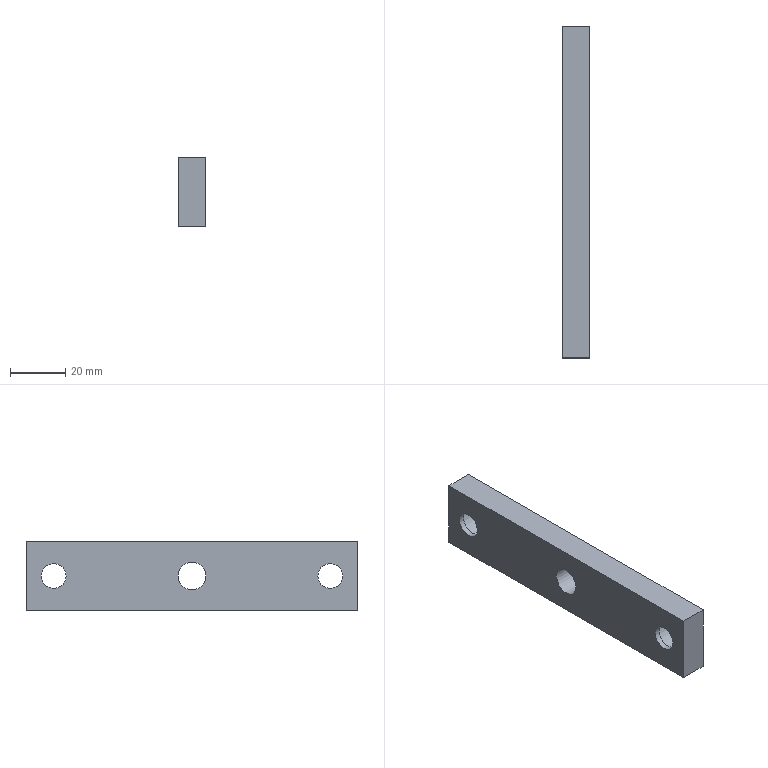Component | NX | FIXTURE_MOUNT_2 | 1 solid | 13 faces | box 10 x 120 x 25 mm | volume 26497 mm3 | plane 8 | cylinder 5 | commonest cylinder face diameters 9 x2 14 x2 10 x1
STEP:
#1=CARTESIAN_POINT('',(0.,0.,0.));
#2=DIRECTION('',(0.,0.,1.));
#3=DIRECTION('',(1.,0.,0.));
#4=AXIS2_PLACEMENT_3D('',#1,#2,#3);
#5=CARTESIAN_POINT('',(746.689,-204.802,-1307.5));
#6=VERTEX_POINT('',#5);
#7=CARTESIAN_POINT('',(746.689,-200.302,-1307.5));
#8=DIRECTION('',(-1.,0.,0.));
#9=DIRECTION('',(0.,-1.,0.));
#10=AXIS2_PLACEMENT_3D('',#7,#8,#9);
#11=CIRCLE('',#10,4.5);
#12=CARTESIAN_POINT('',(756.689,-200.302,-1307.5));
#13=DIRECTION('',(-1.,0.,0.));
#14=DIRECTION('',(0.,-1.,0.));
#15=AXIS2_PLACEMENT_3D('',#12,#13,#14);
#16=CYLINDRICAL_SURFACE('',#15,4.5);
#17=CARTESIAN_POINT('',(0.,10.));
#18=DIRECTION('',(1.,0.));
#19=VECTOR('',#18,1.);
#20=LINE('',#17,#19);
#21=(GEOMETRIC_REPRESENTATION_CONTEXT(2)PARAMETRIC_REPRESENTATION_CONTEXT()REPRESENTATION_CONTEXT('',''));
#22=DEFINITIONAL_REPRESENTATION('',(#20),#21);
#23=PCURVE('',#16,#22);
#24=CARTESIAN_POINT('',(746.689,-150.302,-1307.5));
#25=DIRECTION('',(-1.,0.,0.));
#26=DIRECTION('',(0.,-1.,0.));
#27=AXIS2_PLACEMENT_3D('',#24,#25,#26);
#28=PLANE('',#27);
#29=CARTESIAN_POINT('',(50.,0.));
#30=DIRECTION('',(1.,0.));
#31=AXIS2_PLACEMENT_2D('',#29,#30);
#32=CIRCLE('',#31,4.5);
#33=(GEOMETRIC_REPRESENTATION_CONTEXT(2)PARAMETRIC_REPRESENTATION_CONTEXT()REPRESENTATION_CONTEXT('',''));
#34=DEFINITIONAL_REPRESENTATION('',(#32),#33);
#35=PCURVE('',#28,#34);
#36=SURFACE_CURVE('',#11,(#23,#35),.PCURVE_S1.);
#37=EDGE_CURVE('',#6,#6,#36,.T.);
#38=ORIENTED_EDGE('',*,*,#37,.F.);
#39=CARTESIAN_POINT('',(748.689,-204.802,-1307.5));
#40=VERTEX_POINT('',#39);
#41=CARTESIAN_POINT('',(748.689,-204.802,-1307.5));
#42=CARTESIAN_POINT('',(746.689,-204.802,-1307.5));
#43=B_SPLINE_CURVE_WITH_KNOTS('',1,(#41,#42),.UNSPECIFIED.,.F.,.F.,(2,2),(8.,10.),.PIECEWISE_BEZIER_KNOTS.);
#44=CARTESIAN_POINT('',(0.,0.));
#45=DIRECTION('',(0.,1.));
#46=VECTOR('',#45,1.);
#47=LINE('',#44,#46);
#48=(GEOMETRIC_REPRESENTATION_CONTEXT(2)PARAMETRIC_REPRESENTATION_CONTEXT()REPRESENTATION_CONTEXT('',''));
#49=DEFINITIONAL_REPRESENTATION('',(#47),#48);
#50=PCURVE('',#16,#49);
#51=CARTESIAN_POINT('',(6.283,0.));
#52=DIRECTION('',(0.,1.));
#53=VECTOR('',#52,1.);
#54=LINE('',#51,#53);
#55=(GEOMETRIC_REPRESENTATION_CONTEXT(2)PARAMETRIC_REPRESENTATION_CONTEXT()REPRESENTATION_CONTEXT('',''));
#56=DEFINITIONAL_REPRESENTATION('',(#54),#55);
#57=PCURVE('',#16,#56);
#58=SEAM_CURVE('',#43,(#50,#57),.PCURVE_S1.);
#59=EDGE_CURVE('',#40,#6,#58,.T.);
#60=ORIENTED_EDGE('',*,*,#59,.F.);
#61=CARTESIAN_POINT('',(748.689,-195.802,-1307.5));
#62=VERTEX_POINT('',#61);
#63=CARTESIAN_POINT('',(748.689,-200.302,-1307.5));
#64=DIRECTION('',(-1.,0.,0.));
#65=DIRECTION('',(0.,1.,0.));
#66=AXIS2_PLACEMENT_3D('',#63,#64,#65);
#67=CIRCLE('',#66,4.5);
#68=CARTESIAN_POINT('',(-3.142,8.));
#69=DIRECTION('',(1.,0.));
#70=VECTOR('',#69,1.);
#71=LINE('',#68,#70);
#72=(GEOMETRIC_REPRESENTATION_CONTEXT(2)PARAMETRIC_REPRESENTATION_CONTEXT()REPRESENTATION_CONTEXT('',''));
#73=DEFINITIONAL_REPRESENTATION('',(#71),#72);
#74=PCURVE('',#16,#73);
#75=CARTESIAN_POINT('',(748.689,-200.302,-1307.5));
#76=DIRECTION('',(1.,0.,0.));
#77=DIRECTION('',(0.,1.,0.));
#78=AXIS2_PLACEMENT_3D('',#75,#76,#77);
#79=PLANE('',#78);
#80=CARTESIAN_POINT('',(4.5,0.));
#81=CARTESIAN_POINT('',(4.5,-7.794));
#82=CARTESIAN_POINT('',(-2.25,-3.897));
#83=CARTESIAN_POINT('',(-9.,-0.));
#84=CARTESIAN_POINT('',(-2.25,3.897));
#85=CARTESIAN_POINT('',(4.5,7.794));
#86=CARTESIAN_POINT('',(4.5,0.));
#87=(BOUNDED_CURVE()B_SPLINE_CURVE(2,(#80,#81,#82,#83,#84,#85,#86),.UNSPECIFIED.,.T.,.F.)B_SPLINE_CURVE_WITH_KNOTS((1,2,2,2,2,1),(-2.094,0.,2.094,4.189,6.283,8.378),.UNSPECIFIED.)CURVE()GEOMETRIC_REPRESENTATION_ITEM()RATIONAL_B_SPLINE_CURVE((1.,0.5,1.,0.5,1.,0.5,1.))REPRESENTATION_ITEM(''));
#88=(GEOMETRIC_REPRESENTATION_CONTEXT(2)PARAMETRIC_REPRESENTATION_CONTEXT()REPRESENTATION_CONTEXT('',''));
#89=DEFINITIONAL_REPRESENTATION('',(#87),#88);
#90=PCURVE('',#79,#89);
#91=SURFACE_CURVE('',#67,(#74,#90),.PCURVE_S1.);
#92=EDGE_CURVE('',#40,#62,#91,.T.);
#93=ORIENTED_EDGE('',*,*,#92,.T.);
#94=CARTESIAN_POINT('',(748.689,-200.302,-1307.5));
#95=DIRECTION('',(-1.,0.,0.));
#96=DIRECTION('',(0.,1.,0.));
#97=AXIS2_PLACEMENT_3D('',#94,#95,#96);
#98=CIRCLE('',#97,4.5);
#99=CARTESIAN_POINT('',(3.142,8.));
#100=DIRECTION('',(1.,0.));
#101=VECTOR('',#100,1.);
#102=LINE('',#99,#101);
#103=(GEOMETRIC_REPRESENTATION_CONTEXT(2)PARAMETRIC_REPRESENTATION_CONTEXT()REPRESENTATION_CONTEXT('',''));
#104=DEFINITIONAL_REPRESENTATION('',(#102),#103);
#105=PCURVE('',#16,#104);
#106=CARTESIAN_POINT('',(4.5,0.));
#107=CARTESIAN_POINT('',(4.5,-7.794));
#108=CARTESIAN_POINT('',(-2.25,-3.897));
#109=CARTESIAN_POINT('',(-9.,-0.));
#110=CARTESIAN_POINT('',(-2.25,3.897));
#111=CARTESIAN_POINT('',(4.5,7.794));
#112=CARTESIAN_POINT('',(4.5,0.));
#113=(BOUNDED_CURVE()B_SPLINE_CURVE(2,(#106,#107,#108,#109,#110,#111,#112),.UNSPECIFIED.,.T.,.F.)B_SPLINE_CURVE_WITH_KNOTS((1,2,2,2,2,1),(-2.094,0.,2.094,4.189,6.283,8.378),.UNSPECIFIED.)CURVE()GEOMETRIC_REPRESENTATION_ITEM()RATIONAL_B_SPLINE_CURVE((1.,0.5,1.,0.5,1.,0.5,1.))REPRESENTATION_ITEM(''));
#114=(GEOMETRIC_REPRESENTATION_CONTEXT(2)PARAMETRIC_REPRESENTATION_CONTEXT()REPRESENTATION_CONTEXT('',''));
#115=DEFINITIONAL_REPRESENTATION('',(#113),#114);
#116=PCURVE('',#79,#115);
#117=SURFACE_CURVE('',#98,(#105,#116),.PCURVE_S1.);
#118=EDGE_CURVE('',#62,#40,#117,.T.);
#119=ORIENTED_EDGE('',*,*,#118,.T.);
#120=ORIENTED_EDGE('',*,*,#59,.T.);
#121=EDGE_LOOP('',(#38,#60,#93,#119,#120));
#122=FACE_BOUND('',#121,.F.);
#123=ADVANCED_FACE('',(#122),#16,.F.);
#124=CARTESIAN_POINT('',(746.689,-95.802,-1307.5));
#125=VERTEX_POINT('',#124);
#126=CARTESIAN_POINT('',(746.689,-100.302,-1307.5));
#127=DIRECTION('',(1.,0.,0.));
#128=DIRECTION('',(0.,1.,0.));
#129=AXIS2_PLACEMENT_3D('',#126,#127,#128);
#130=CIRCLE('',#129,4.5);
#131=CARTESIAN_POINT('',(756.689,-100.302,-1307.5));
#132=DIRECTION('',(-1.,0.,0.));
#133=DIRECTION('',(0.,-1.,0.));
#134=AXIS2_PLACEMENT_3D('',#131,#132,#133);
#135=CYLINDRICAL_SURFACE('',#134,4.5);
#136=CARTESIAN_POINT('',(9.425,10.));
#137=DIRECTION('',(-1.,0.));
#138=VECTOR('',#137,1.);
#139=LINE('',#136,#138);
#140=(GEOMETRIC_REPRESENTATION_CONTEXT(2)PARAMETRIC_REPRESENTATION_CONTEXT()REPRESENTATION_CONTEXT('',''));
#141=DEFINITIONAL_REPRESENTATION('',(#139),#140);
#142=PCURVE('',#135,#141);
#143=CARTESIAN_POINT('',(-54.5,0.));
#144=CARTESIAN_POINT('',(-54.5,7.794));
#145=CARTESIAN_POINT('',(-47.75,3.897));
#146=CARTESIAN_POINT('',(-41.,0.));
#147=CARTESIAN_POINT('',(-47.75,-3.897));
#148=CARTESIAN_POINT('',(-54.5,-7.794));
#149=CARTESIAN_POINT('',(-54.5,0.));
#150=(BOUNDED_CURVE()B_SPLINE_CURVE(2,(#143,#144,#145,#146,#147,#148,#149),.UNSPECIFIED.,.T.,.F.)B_SPLINE_CURVE_WITH_KNOTS((1,2,2,2,2,1),(-2.094,0.,2.094,4.189,6.283,8.378),.UNSPECIFIED.)CURVE()GEOMETRIC_REPRESENTATION_ITEM()RATIONAL_B_SPLINE_CURVE((1.,0.5,1.,0.5,1.,0.5,1.))REPRESENTATION_ITEM(''));
#151=(GEOMETRIC_REPRESENTATION_CONTEXT(2)PARAMETRIC_REPRESENTATION_CONTEXT()REPRESENTATION_CONTEXT('',''));
#152=DEFINITIONAL_REPRESENTATION('',(#150),#151);
#153=PCURVE('',#28,#152);
#154=SURFACE_CURVE('',#130,(#142,#153),.PCURVE_S1.);
#155=EDGE_CURVE('',#125,#125,#154,.T.);
#156=ORIENTED_EDGE('',*,*,#155,.T.);
#157=CARTESIAN_POINT('',(748.689,-95.802,-1307.5));
#158=VERTEX_POINT('',#157);
#159=CARTESIAN_POINT('',(748.689,-95.802,-1307.5));
#160=CARTESIAN_POINT('',(746.689,-95.802,-1307.5));
#161=B_SPLINE_CURVE_WITH_KNOTS('',1,(#159,#160),.UNSPECIFIED.,.F.,.F.,(2,2),(8.,10.),.PIECEWISE_BEZIER_KNOTS.);
#162=CARTESIAN_POINT('',(3.142,0.));
#163=DIRECTION('',(0.,1.));
#164=VECTOR('',#163,1.);
#165=LINE('',#162,#164);
#166=(GEOMETRIC_REPRESENTATION_CONTEXT(2)PARAMETRIC_REPRESENTATION_CONTEXT()REPRESENTATION_CONTEXT('',''));
#167=DEFINITIONAL_REPRESENTATION('',(#165),#166);
#168=PCURVE('',#135,#167);
#169=CARTESIAN_POINT('',(9.425,0.));
#170=DIRECTION('',(0.,1.));
#171=VECTOR('',#170,1.);
#172=LINE('',#169,#171);
#173=(GEOMETRIC_REPRESENTATION_CONTEXT(2)PARAMETRIC_REPRESENTATION_CONTEXT()REPRESENTATION_CONTEXT('',''));
#174=DEFINITIONAL_REPRESENTATION('',(#172),#173);
#175=PCURVE('',#135,#174);
#176=SEAM_CURVE('',#161,(#168,#175),.PCURVE_S1.);
#177=EDGE_CURVE('',#158,#125,#176,.T.);
#178=ORIENTED_EDGE('',*,*,#177,.F.);
#179=CARTESIAN_POINT('',(748.689,-100.302,-1307.5));
#180=DIRECTION('',(1.,0.,0.));
#181=DIRECTION('',(0.,1.,0.));
#182=AXIS2_PLACEMENT_3D('',#179,#180,#181);
#183=CIRCLE('',#182,4.5);
#184=CARTESIAN_POINT('',(9.425,8.));
#185=DIRECTION('',(-1.,0.));
#186=VECTOR('',#185,1.);
#187=LINE('',#184,#186);
#188=(GEOMETRIC_REPRESENTATION_CONTEXT(2)PARAMETRIC_REPRESENTATION_CONTEXT()REPRESENTATION_CONTEXT('',''));
#189=DEFINITIONAL_REPRESENTATION('',(#187),#188);
#190=PCURVE('',#135,#189);
#191=CARTESIAN_POINT('',(748.689,-100.302,-1307.5));
#192=DIRECTION('',(1.,0.,0.));
#193=DIRECTION('',(0.,1.,0.));
#194=AXIS2_PLACEMENT_3D('',#191,#192,#193);
#195=PLANE('',#194);
#196=CARTESIAN_POINT('',(0.,0.));
#197=DIRECTION('',(1.,0.));
#198=AXIS2_PLACEMENT_2D('',#196,#197);
#199=CIRCLE('',#198,4.5);
#200=(GEOMETRIC_REPRESENTATION_CONTEXT(2)PARAMETRIC_REPRESENTATION_CONTEXT()REPRESENTATION_CONTEXT('',''));
#201=DEFINITIONAL_REPRESENTATION('',(#199),#200);
#202=PCURVE('',#195,#201);
#203=SURFACE_CURVE('',#183,(#190,#202),.PCURVE_S1.);
#204=EDGE_CURVE('',#158,#158,#203,.T.);
#205=ORIENTED_EDGE('',*,*,#204,.F.);
#206=ORIENTED_EDGE('',*,*,#177,.T.);
#207=EDGE_LOOP('',(#156,#178,#205,#206));
#208=FACE_BOUND('',#207,.F.);
#209=ADVANCED_FACE('',(#208),#135,.F.);
#210=CARTESIAN_POINT('',(746.689,-210.302,-1295.));
#211=VERTEX_POINT('',#210);
#212=CARTESIAN_POINT('',(746.689,-210.302,-1320.));
#213=VERTEX_POINT('',#212);
#214=CARTESIAN_POINT('',(746.689,-210.302,-1295.));
#215=DIRECTION('',(0.,0.,-1.));
#216=VECTOR('',#215,1.);
#217=LINE('',#214,#216);
#218=CARTESIAN_POINT('',(756.689,-210.302,-1295.));
#219=DIRECTION('',(0.,1.,0.));
#220=DIRECTION('',(-1.,0.,0.));
#221=AXIS2_PLACEMENT_3D('',#218,#219,#220);
#222=PLANE('',#221);
#223=CARTESIAN_POINT('',(10.,0.));
#224=DIRECTION('',(0.,-1.));
#225=VECTOR('',#224,1.);
#226=LINE('',#223,#225);
#227=(GEOMETRIC_REPRESENTATION_CONTEXT(2)PARAMETRIC_REPRESENTATION_CONTEXT()REPRESENTATION_CONTEXT('',''));
#228=DEFINITIONAL_REPRESENTATION('',(#226),#227);
#229=PCURVE('',#222,#228);
#230=CARTESIAN_POINT('',(60.,12.5));
#231=DIRECTION('',(0.,-1.));
#232=VECTOR('',#231,1.);
#233=LINE('',#230,#232);
#234=(GEOMETRIC_REPRESENTATION_CONTEXT(2)PARAMETRIC_REPRESENTATION_CONTEXT()REPRESENTATION_CONTEXT('',''));
#235=DEFINITIONAL_REPRESENTATION('',(#233),#234);
#236=PCURVE('',#28,#235);
#237=SURFACE_CURVE('',#217,(#229,#236),.PCURVE_S1.);
#238=EDGE_CURVE('',#211,#213,#237,.T.);
#239=ORIENTED_EDGE('',*,*,#238,.T.);
#240=CARTESIAN_POINT('',(756.689,-210.302,-1320.));
#241=VERTEX_POINT('',#240);
#242=CARTESIAN_POINT('',(756.689,-210.302,-1320.));
#243=DIRECTION('',(-1.,0.,0.));
#244=VECTOR('',#243,1.);
#245=LINE('',#242,#244);
#246=CARTESIAN_POINT('',(0.,-25.));
#247=DIRECTION('',(1.,0.));
#248=VECTOR('',#247,1.);
#249=LINE('',#246,#248);
#250=(GEOMETRIC_REPRESENTATION_CONTEXT(2)PARAMETRIC_REPRESENTATION_CONTEXT()REPRESENTATION_CONTEXT('',''));
#251=DEFINITIONAL_REPRESENTATION('',(#249),#250);
#252=PCURVE('',#222,#251);
#253=CARTESIAN_POINT('',(756.689,-210.302,-1320.));
#254=DIRECTION('',(0.,0.,1.));
#255=DIRECTION('',(1.,0.,0.));
#256=AXIS2_PLACEMENT_3D('',#253,#254,#255);
#257=PLANE('',#256);
#258=CARTESIAN_POINT('',(0.,0.));
#259=DIRECTION('',(-1.,0.));
#260=VECTOR('',#259,1.);
#261=LINE('',#258,#260);
#262=(GEOMETRIC_REPRESENTATION_CONTEXT(2)PARAMETRIC_REPRESENTATION_CONTEXT()REPRESENTATION_CONTEXT('',''));
#263=DEFINITIONAL_REPRESENTATION('',(#261),#262);
#264=PCURVE('',#257,#263);
#265=SURFACE_CURVE('',#245,(#252,#264),.PCURVE_S1.);
#266=EDGE_CURVE('',#241,#213,#265,.T.);
#267=ORIENTED_EDGE('',*,*,#266,.F.);
#268=CARTESIAN_POINT('',(756.689,-210.302,-1295.));
#269=VERTEX_POINT('',#268);
#270=CARTESIAN_POINT('',(756.689,-210.302,-1295.));
#271=DIRECTION('',(0.,0.,-1.));
#272=VECTOR('',#271,1.);
#273=LINE('',#270,#272);
#274=CARTESIAN_POINT('',(0.,0.));
#275=DIRECTION('',(0.,-1.));
#276=VECTOR('',#275,1.);
#277=LINE('',#274,#276);
#278=(GEOMETRIC_REPRESENTATION_CONTEXT(2)PARAMETRIC_REPRESENTATION_CONTEXT()REPRESENTATION_CONTEXT('',''));
#279=DEFINITIONAL_REPRESENTATION('',(#277),#278);
#280=PCURVE('',#222,#279);
#281=CARTESIAN_POINT('',(756.689,-150.302,-1307.5));
#282=DIRECTION('',(-1.,0.,0.));
#283=DIRECTION('',(0.,-1.,0.));
#284=AXIS2_PLACEMENT_3D('',#281,#282,#283);
#285=PLANE('',#284);
#286=CARTESIAN_POINT('',(60.,12.5));
#287=DIRECTION('',(0.,-1.));
#288=VECTOR('',#287,1.);
#289=LINE('',#286,#288);
#290=(GEOMETRIC_REPRESENTATION_CONTEXT(2)PARAMETRIC_REPRESENTATION_CONTEXT()REPRESENTATION_CONTEXT('',''));
#291=DEFINITIONAL_REPRESENTATION('',(#289),#290);
#292=PCURVE('',#285,#291);
#293=SURFACE_CURVE('',#273,(#280,#292),.PCURVE_S1.);
#294=EDGE_CURVE('',#269,#241,#293,.T.);
#295=ORIENTED_EDGE('',*,*,#294,.F.);
#296=CARTESIAN_POINT('',(756.689,-210.302,-1295.));
#297=DIRECTION('',(-1.,0.,0.));
#298=VECTOR('',#297,1.);
#299=LINE('',#296,#298);
#300=CARTESIAN_POINT('',(0.,0.));
#301=DIRECTION('',(1.,0.));
#302=VECTOR('',#301,1.);
#303=LINE('',#300,#302);
#304=(GEOMETRIC_REPRESENTATION_CONTEXT(2)PARAMETRIC_REPRESENTATION_CONTEXT()REPRESENTATION_CONTEXT('',''));
#305=DEFINITIONAL_REPRESENTATION('',(#303),#304);
#306=PCURVE('',#222,#305);
#307=CARTESIAN_POINT('',(756.689,-90.302,-1295.));
#308=DIRECTION('',(0.,0.,-1.));
#309=DIRECTION('',(-1.,0.,0.));
#310=AXIS2_PLACEMENT_3D('',#307,#308,#309);
#311=PLANE('',#310);
#312=CARTESIAN_POINT('',(0.,-120.));
#313=DIRECTION('',(1.,0.));
#314=VECTOR('',#313,1.);
#315=LINE('',#312,#314);
#316=(GEOMETRIC_REPRESENTATION_CONTEXT(2)PARAMETRIC_REPRESENTATION_CONTEXT()REPRESENTATION_CONTEXT('',''));
#317=DEFINITIONAL_REPRESENTATION('',(#315),#316);
#318=PCURVE('',#311,#317);
#319=SURFACE_CURVE('',#299,(#306,#318),.PCURVE_S1.);
#320=EDGE_CURVE('',#269,#211,#319,.T.);
#321=ORIENTED_EDGE('',*,*,#320,.T.);
#322=EDGE_LOOP('',(#239,#267,#295,#321));
#323=FACE_BOUND('',#322,.T.);
#324=ADVANCED_FACE('',(#323),#222,.F.);
#325=CARTESIAN_POINT('',(746.689,-90.302,-1320.));
#326=VERTEX_POINT('',#325);
#327=CARTESIAN_POINT('',(746.689,-210.302,-1320.));
#328=DIRECTION('',(0.,1.,0.));
#329=VECTOR('',#328,1.);
#330=LINE('',#327,#329);
#331=CARTESIAN_POINT('',(-10.,0.));
#332=DIRECTION('',(0.,1.));
#333=VECTOR('',#332,1.);
#334=LINE('',#331,#333);
#335=(GEOMETRIC_REPRESENTATION_CONTEXT(2)PARAMETRIC_REPRESENTATION_CONTEXT()REPRESENTATION_CONTEXT('',''));
#336=DEFINITIONAL_REPRESENTATION('',(#334),#335);
#337=PCURVE('',#257,#336);
#338=CARTESIAN_POINT('',(60.,-12.5));
#339=DIRECTION('',(-1.,0.));
#340=VECTOR('',#339,1.);
#341=LINE('',#338,#340);
#342=(GEOMETRIC_REPRESENTATION_CONTEXT(2)PARAMETRIC_REPRESENTATION_CONTEXT()REPRESENTATION_CONTEXT('',''));
#343=DEFINITIONAL_REPRESENTATION('',(#341),#342);
#344=PCURVE('',#28,#343);
#345=SURFACE_CURVE('',#330,(#337,#344),.PCURVE_S1.);
#346=EDGE_CURVE('',#213,#326,#345,.T.);
#347=ORIENTED_EDGE('',*,*,#346,.T.);
#348=CARTESIAN_POINT('',(756.689,-90.302,-1320.));
#349=VERTEX_POINT('',#348);
#350=CARTESIAN_POINT('',(756.689,-90.302,-1320.));
#351=DIRECTION('',(-1.,0.,0.));
#352=VECTOR('',#351,1.);
#353=LINE('',#350,#352);
#354=CARTESIAN_POINT('',(0.,120.));
#355=DIRECTION('',(-1.,0.));
#356=VECTOR('',#355,1.);
#357=LINE('',#354,#356);
#358=(GEOMETRIC_REPRESENTATION_CONTEXT(2)PARAMETRIC_REPRESENTATION_CONTEXT()REPRESENTATION_CONTEXT('',''));
#359=DEFINITIONAL_REPRESENTATION('',(#357),#358);
#360=PCURVE('',#257,#359);
#361=CARTESIAN_POINT('',(756.689,-90.302,-1320.));
#362=DIRECTION('',(0.,-1.,0.));
#363=DIRECTION('',(1.,0.,0.));
#364=AXIS2_PLACEMENT_3D('',#361,#362,#363);
#365=PLANE('',#364);
#366=CARTESIAN_POINT('',(0.,0.));
#367=DIRECTION('',(-1.,0.));
#368=VECTOR('',#367,1.);
#369=LINE('',#366,#368);
#370=(GEOMETRIC_REPRESENTATION_CONTEXT(2)PARAMETRIC_REPRESENTATION_CONTEXT()REPRESENTATION_CONTEXT('',''));
#371=DEFINITIONAL_REPRESENTATION('',(#369),#370);
#372=PCURVE('',#365,#371);
#373=SURFACE_CURVE('',#353,(#360,#372),.PCURVE_S1.);
#374=EDGE_CURVE('',#349,#326,#373,.T.);
#375=ORIENTED_EDGE('',*,*,#374,.F.);
#376=CARTESIAN_POINT('',(756.689,-210.302,-1320.));
#377=DIRECTION('',(0.,1.,0.));
#378=VECTOR('',#377,1.);
#379=LINE('',#376,#378);
#380=CARTESIAN_POINT('',(0.,0.));
#381=DIRECTION('',(0.,1.));
#382=VECTOR('',#381,1.);
#383=LINE('',#380,#382);
#384=(GEOMETRIC_REPRESENTATION_CONTEXT(2)PARAMETRIC_REPRESENTATION_CONTEXT()REPRESENTATION_CONTEXT('',''));
#385=DEFINITIONAL_REPRESENTATION('',(#383),#384);
#386=PCURVE('',#257,#385);
#387=CARTESIAN_POINT('',(60.,-12.5));
#388=DIRECTION('',(-1.,0.));
#389=VECTOR('',#388,1.);
#390=LINE('',#387,#389);
#391=(GEOMETRIC_REPRESENTATION_CONTEXT(2)PARAMETRIC_REPRESENTATION_CONTEXT()REPRESENTATION_CONTEXT('',''));
#392=DEFINITIONAL_REPRESENTATION('',(#390),#391);
#393=PCURVE('',#285,#392);
#394=SURFACE_CURVE('',#379,(#386,#393),.PCURVE_S1.);
#395=EDGE_CURVE('',#241,#349,#394,.T.);
#396=ORIENTED_EDGE('',*,*,#395,.F.);
#397=ORIENTED_EDGE('',*,*,#266,.T.);
#398=EDGE_LOOP('',(#347,#375,#396,#397));
#399=FACE_BOUND('',#398,.T.);
#400=ADVANCED_FACE('',(#399),#257,.F.);
#401=CARTESIAN_POINT('',(746.689,-90.302,-1295.));
#402=VERTEX_POINT('',#401);
#403=CARTESIAN_POINT('',(746.689,-90.302,-1320.));
#404=DIRECTION('',(0.,0.,1.));
#405=VECTOR('',#404,1.);
#406=LINE('',#403,#405);
#407=CARTESIAN_POINT('',(-10.,0.));
#408=DIRECTION('',(0.,1.));
#409=VECTOR('',#408,1.);
#410=LINE('',#407,#409);
#411=(GEOMETRIC_REPRESENTATION_CONTEXT(2)PARAMETRIC_REPRESENTATION_CONTEXT()REPRESENTATION_CONTEXT('',''));
#412=DEFINITIONAL_REPRESENTATION('',(#410),#411);
#413=PCURVE('',#365,#412);
#414=CARTESIAN_POINT('',(-60.,-12.5));
#415=DIRECTION('',(0.,1.));
#416=VECTOR('',#415,1.);
#417=LINE('',#414,#416);
#418=(GEOMETRIC_REPRESENTATION_CONTEXT(2)PARAMETRIC_REPRESENTATION_CONTEXT()REPRESENTATION_CONTEXT('',''));
#419=DEFINITIONAL_REPRESENTATION('',(#417),#418);
#420=PCURVE('',#28,#419);
#421=SURFACE_CURVE('',#406,(#413,#420),.PCURVE_S1.);
#422=EDGE_CURVE('',#326,#402,#421,.T.);
#423=ORIENTED_EDGE('',*,*,#422,.T.);
#424=CARTESIAN_POINT('',(756.689,-90.302,-1295.));
#425=VERTEX_POINT('',#424);
#426=CARTESIAN_POINT('',(756.689,-90.302,-1295.));
#427=DIRECTION('',(-1.,0.,0.));
#428=VECTOR('',#427,1.);
#429=LINE('',#426,#428);
#430=CARTESIAN_POINT('',(0.,25.));
#431=DIRECTION('',(-1.,0.));
#432=VECTOR('',#431,1.);
#433=LINE('',#430,#432);
#434=(GEOMETRIC_REPRESENTATION_CONTEXT(2)PARAMETRIC_REPRESENTATION_CONTEXT()REPRESENTATION_CONTEXT('',''));
#435=DEFINITIONAL_REPRESENTATION('',(#433),#434);
#436=PCURVE('',#365,#435);
#437=CARTESIAN_POINT('',(0.,0.));
#438=DIRECTION('',(1.,0.));
#439=VECTOR('',#438,1.);
#440=LINE('',#437,#439);
#441=(GEOMETRIC_REPRESENTATION_CONTEXT(2)PARAMETRIC_REPRESENTATION_CONTEXT()REPRESENTATION_CONTEXT('',''));
#442=DEFINITIONAL_REPRESENTATION('',(#440),#441);
#443=PCURVE('',#311,#442);
#444=SURFACE_CURVE('',#429,(#436,#443),.PCURVE_S1.);
#445=EDGE_CURVE('',#425,#402,#444,.T.);
#446=ORIENTED_EDGE('',*,*,#445,.F.);
#447=CARTESIAN_POINT('',(756.689,-90.302,-1320.));
#448=DIRECTION('',(0.,0.,1.));
#449=VECTOR('',#448,1.);
#450=LINE('',#447,#449);
#451=CARTESIAN_POINT('',(0.,0.));
#452=DIRECTION('',(0.,1.));
#453=VECTOR('',#452,1.);
#454=LINE('',#451,#453);
#455=(GEOMETRIC_REPRESENTATION_CONTEXT(2)PARAMETRIC_REPRESENTATION_CONTEXT()REPRESENTATION_CONTEXT('',''));
#456=DEFINITIONAL_REPRESENTATION('',(#454),#455);
#457=PCURVE('',#365,#456);
#458=CARTESIAN_POINT('',(-60.,-12.5));
#459=DIRECTION('',(0.,1.));
#460=VECTOR('',#459,1.);
#461=LINE('',#458,#460);
#462=(GEOMETRIC_REPRESENTATION_CONTEXT(2)PARAMETRIC_REPRESENTATION_CONTEXT()REPRESENTATION_CONTEXT('',''));
#463=DEFINITIONAL_REPRESENTATION('',(#461),#462);
#464=PCURVE('',#285,#463);
#465=SURFACE_CURVE('',#450,(#457,#464),.PCURVE_S1.);
#466=EDGE_CURVE('',#349,#425,#465,.T.);
#467=ORIENTED_EDGE('',*,*,#466,.F.);
#468=ORIENTED_EDGE('',*,*,#374,.T.);
#469=EDGE_LOOP('',(#423,#446,#467,#468));
#470=FACE_BOUND('',#469,.T.);
#471=ADVANCED_FACE('',(#470),#365,.F.);
#472=CARTESIAN_POINT('',(756.689,-155.302,-1307.5));
#473=VERTEX_POINT('',#472);
#474=CARTESIAN_POINT('',(756.689,-150.302,-1307.5));
#475=DIRECTION('',(-1.,0.,0.));
#476=DIRECTION('',(0.,-1.,0.));
#477=AXIS2_PLACEMENT_3D('',#474,#475,#476);
#478=CIRCLE('',#477,5.);
#479=CARTESIAN_POINT('',(756.689,-150.302,-1307.5));
#480=DIRECTION('',(-1.,0.,0.));
#481=DIRECTION('',(0.,-1.,0.));
#482=AXIS2_PLACEMENT_3D('',#479,#480,#481);
#483=CYLINDRICAL_SURFACE('',#482,5.);
#484=CARTESIAN_POINT('',(0.,0.));
#485=DIRECTION('',(1.,0.));
#486=VECTOR('',#485,1.);
#487=LINE('',#484,#486);
#488=(GEOMETRIC_REPRESENTATION_CONTEXT(2)PARAMETRIC_REPRESENTATION_CONTEXT()REPRESENTATION_CONTEXT('',''));
#489=DEFINITIONAL_REPRESENTATION('',(#487),#488);
#490=PCURVE('',#483,#489);
#491=CARTESIAN_POINT('',(0.,0.));
#492=DIRECTION('',(1.,0.));
#493=AXIS2_PLACEMENT_2D('',#491,#492);
#494=CIRCLE('',#493,5.);
#495=(GEOMETRIC_REPRESENTATION_CONTEXT(2)PARAMETRIC_REPRESENTATION_CONTEXT()REPRESENTATION_CONTEXT('',''));
#496=DEFINITIONAL_REPRESENTATION('',(#494),#495);
#497=PCURVE('',#285,#496);
#498=SURFACE_CURVE('',#478,(#490,#497),.PCURVE_S1.);
#499=EDGE_CURVE('',#473,#473,#498,.T.);
#500=ORIENTED_EDGE('',*,*,#499,.T.);
#501=CARTESIAN_POINT('',(746.689,-155.302,-1307.5));
#502=VERTEX_POINT('',#501);
#503=CARTESIAN_POINT('',(756.689,-155.302,-1307.5));
#504=CARTESIAN_POINT('',(746.689,-155.302,-1307.5));
#505=B_SPLINE_CURVE_WITH_KNOTS('',1,(#503,#504),.UNSPECIFIED.,.F.,.F.,(2,2),(0.,10.),.PIECEWISE_BEZIER_KNOTS.);
#506=CARTESIAN_POINT('',(6.283,0.));
#507=DIRECTION('',(0.,1.));
#508=VECTOR('',#507,1.);
#509=LINE('',#506,#508);
#510=(GEOMETRIC_REPRESENTATION_CONTEXT(2)PARAMETRIC_REPRESENTATION_CONTEXT()REPRESENTATION_CONTEXT('',''));
#511=DEFINITIONAL_REPRESENTATION('',(#509),#510);
#512=PCURVE('',#483,#511);
#513=CARTESIAN_POINT('',(0.,0.));
#514=DIRECTION('',(0.,1.));
#515=VECTOR('',#514,1.);
#516=LINE('',#513,#515);
#517=(GEOMETRIC_REPRESENTATION_CONTEXT(2)PARAMETRIC_REPRESENTATION_CONTEXT()REPRESENTATION_CONTEXT('',''));
#518=DEFINITIONAL_REPRESENTATION('',(#516),#517);
#519=PCURVE('',#483,#518);
#520=SEAM_CURVE('',#505,(#512,#519),.PCURVE_S1.);
#521=EDGE_CURVE('',#473,#502,#520,.T.);
#522=ORIENTED_EDGE('',*,*,#521,.T.);
#523=CARTESIAN_POINT('',(746.689,-150.302,-1307.5));
#524=DIRECTION('',(-1.,0.,0.));
#525=DIRECTION('',(0.,-1.,0.));
#526=AXIS2_PLACEMENT_3D('',#523,#524,#525);
#527=CIRCLE('',#526,5.);
#528=CARTESIAN_POINT('',(0.,10.));
#529=DIRECTION('',(1.,0.));
#530=VECTOR('',#529,1.);
#531=LINE('',#528,#530);
#532=(GEOMETRIC_REPRESENTATION_CONTEXT(2)PARAMETRIC_REPRESENTATION_CONTEXT()REPRESENTATION_CONTEXT('',''));
#533=DEFINITIONAL_REPRESENTATION('',(#531),#532);
#534=PCURVE('',#483,#533);
#535=CARTESIAN_POINT('',(0.,0.));
#536=DIRECTION('',(1.,0.));
#537=AXIS2_PLACEMENT_2D('',#535,#536);
#538=CIRCLE('',#537,5.);
#539=(GEOMETRIC_REPRESENTATION_CONTEXT(2)PARAMETRIC_REPRESENTATION_CONTEXT()REPRESENTATION_CONTEXT('',''));
#540=DEFINITIONAL_REPRESENTATION('',(#538),#539);
#541=PCURVE('',#28,#540);
#542=SURFACE_CURVE('',#527,(#534,#541),.PCURVE_S1.);
#543=EDGE_CURVE('',#502,#502,#542,.T.);
#544=ORIENTED_EDGE('',*,*,#543,.F.);
#545=ORIENTED_EDGE('',*,*,#521,.F.);
#546=EDGE_LOOP('',(#500,#522,#544,#545));
#547=FACE_BOUND('',#546,.F.);
#548=ADVANCED_FACE('',(#547),#483,.F.);
#549=CARTESIAN_POINT('',(746.689,-90.302,-1295.));
#550=DIRECTION('',(0.,-1.,0.));
#551=VECTOR('',#550,1.);
#552=LINE('',#549,#551);
#553=CARTESIAN_POINT('',(10.,0.));
#554=DIRECTION('',(0.,-1.));
#555=VECTOR('',#554,1.);
#556=LINE('',#553,#555);
#557=(GEOMETRIC_REPRESENTATION_CONTEXT(2)PARAMETRIC_REPRESENTATION_CONTEXT()REPRESENTATION_CONTEXT('',''));
#558=DEFINITIONAL_REPRESENTATION('',(#556),#557);
#559=PCURVE('',#311,#558);
#560=CARTESIAN_POINT('',(-60.,12.5));
#561=DIRECTION('',(1.,0.));
#562=VECTOR('',#561,1.);
#563=LINE('',#560,#562);
#564=(GEOMETRIC_REPRESENTATION_CONTEXT(2)PARAMETRIC_REPRESENTATION_CONTEXT()REPRESENTATION_CONTEXT('',''));
#565=DEFINITIONAL_REPRESENTATION('',(#563),#564);
#566=PCURVE('',#28,#565);
#567=SURFACE_CURVE('',#552,(#559,#566),.PCURVE_S1.);
#568=EDGE_CURVE('',#402,#211,#567,.T.);
#569=ORIENTED_EDGE('',*,*,#568,.T.);
#570=ORIENTED_EDGE('',*,*,#320,.F.);
#571=CARTESIAN_POINT('',(756.689,-90.302,-1295.));
#572=DIRECTION('',(0.,-1.,0.));
#573=VECTOR('',#572,1.);
#574=LINE('',#571,#573);
#575=CARTESIAN_POINT('',(0.,0.));
#576=DIRECTION('',(0.,-1.));
#577=VECTOR('',#576,1.);
#578=LINE('',#575,#577);
#579=(GEOMETRIC_REPRESENTATION_CONTEXT(2)PARAMETRIC_REPRESENTATION_CONTEXT()REPRESENTATION_CONTEXT('',''));
#580=DEFINITIONAL_REPRESENTATION('',(#578),#579);
#581=PCURVE('',#311,#580);
#582=CARTESIAN_POINT('',(-60.,12.5));
#583=DIRECTION('',(1.,0.));
#584=VECTOR('',#583,1.);
#585=LINE('',#582,#584);
#586=(GEOMETRIC_REPRESENTATION_CONTEXT(2)PARAMETRIC_REPRESENTATION_CONTEXT()REPRESENTATION_CONTEXT('',''));
#587=DEFINITIONAL_REPRESENTATION('',(#585),#586);
#588=PCURVE('',#285,#587);
#589=SURFACE_CURVE('',#574,(#581,#588),.PCURVE_S1.);
#590=EDGE_CURVE('',#425,#269,#589,.T.);
#591=ORIENTED_EDGE('',*,*,#590,.F.);
#592=ORIENTED_EDGE('',*,*,#445,.T.);
#593=EDGE_LOOP('',(#569,#570,#591,#592));
#594=FACE_BOUND('',#593,.T.);
#595=ADVANCED_FACE('',(#594),#311,.F.);
#596=CARTESIAN_POINT('',(756.689,-193.302,-1307.5));
#597=VERTEX_POINT('',#596);
#598=CARTESIAN_POINT('',(756.689,-200.302,-1307.5));
#599=DIRECTION('',(1.,0.,0.));
#600=DIRECTION('',(0.,1.,0.));
#601=AXIS2_PLACEMENT_3D('',#598,#599,#600);
#602=CIRCLE('',#601,7.);
#603=CARTESIAN_POINT('',(43.,0.));
#604=CARTESIAN_POINT('',(43.,12.124));
#605=CARTESIAN_POINT('',(53.5,6.062));
#606=CARTESIAN_POINT('',(64.,0.));
#607=CARTESIAN_POINT('',(53.5,-6.062));
#608=CARTESIAN_POINT('',(43.,-12.124));
#609=CARTESIAN_POINT('',(43.,0.));
#610=(BOUNDED_CURVE()B_SPLINE_CURVE(2,(#603,#604,#605,#606,#607,#608,#609),.UNSPECIFIED.,.T.,.F.)B_SPLINE_CURVE_WITH_KNOTS((1,2,2,2,2,1),(-2.094,0.,2.094,4.189,6.283,8.378),.UNSPECIFIED.)CURVE()GEOMETRIC_REPRESENTATION_ITEM()RATIONAL_B_SPLINE_CURVE((1.,0.5,1.,0.5,1.,0.5,1.))REPRESENTATION_ITEM(''));
#611=(GEOMETRIC_REPRESENTATION_CONTEXT(2)PARAMETRIC_REPRESENTATION_CONTEXT()REPRESENTATION_CONTEXT('',''));
#612=DEFINITIONAL_REPRESENTATION('',(#610),#611);
#613=PCURVE('',#285,#612);
#614=CARTESIAN_POINT('',(748.689,-200.302,-1307.5));
#615=DIRECTION('',(1.,0.,0.));
#616=DIRECTION('',(0.,1.,0.));
#617=AXIS2_PLACEMENT_3D('',#614,#615,#616);
#618=CYLINDRICAL_SURFACE('',#617,7.);
#619=CARTESIAN_POINT('',(0.,8.));
#620=DIRECTION('',(1.,0.));
#621=VECTOR('',#620,1.);
#622=LINE('',#619,#621);
#623=(GEOMETRIC_REPRESENTATION_CONTEXT(2)PARAMETRIC_REPRESENTATION_CONTEXT()REPRESENTATION_CONTEXT('',''));
#624=DEFINITIONAL_REPRESENTATION('',(#622),#623);
#625=PCURVE('',#618,#624);
#626=SURFACE_CURVE('',#602,(#613,#625),.PCURVE_S1.);
#627=EDGE_CURVE('',#597,#597,#626,.T.);
#628=ORIENTED_EDGE('',*,*,#627,.F.);
#629=EDGE_LOOP('',(#628));
#630=FACE_BOUND('',#629,.T.);
#631=CARTESIAN_POINT('',(756.689,-93.302,-1307.5));
#632=VERTEX_POINT('',#631);
#633=CARTESIAN_POINT('',(756.689,-100.302,-1307.5));
#634=DIRECTION('',(1.,0.,0.));
#635=DIRECTION('',(0.,1.,0.));
#636=AXIS2_PLACEMENT_3D('',#633,#634,#635);
#637=CIRCLE('',#636,7.);
#638=CARTESIAN_POINT('',(-57.,0.));
#639=CARTESIAN_POINT('',(-57.,12.124));
#640=CARTESIAN_POINT('',(-46.5,6.062));
#641=CARTESIAN_POINT('',(-36.,0.));
#642=CARTESIAN_POINT('',(-46.5,-6.062));
#643=CARTESIAN_POINT('',(-57.,-12.124));
#644=CARTESIAN_POINT('',(-57.,0.));
#645=(BOUNDED_CURVE()B_SPLINE_CURVE(2,(#638,#639,#640,#641,#642,#643,#644),.UNSPECIFIED.,.T.,.F.)B_SPLINE_CURVE_WITH_KNOTS((1,2,2,2,2,1),(-2.094,0.,2.094,4.189,6.283,8.378),.UNSPECIFIED.)CURVE()GEOMETRIC_REPRESENTATION_ITEM()RATIONAL_B_SPLINE_CURVE((1.,0.5,1.,0.5,1.,0.5,1.))REPRESENTATION_ITEM(''));
#646=(GEOMETRIC_REPRESENTATION_CONTEXT(2)PARAMETRIC_REPRESENTATION_CONTEXT()REPRESENTATION_CONTEXT('',''));
#647=DEFINITIONAL_REPRESENTATION('',(#645),#646);
#648=PCURVE('',#285,#647);
#649=CARTESIAN_POINT('',(748.689,-100.302,-1307.5));
#650=DIRECTION('',(1.,0.,0.));
#651=DIRECTION('',(0.,1.,0.));
#652=AXIS2_PLACEMENT_3D('',#649,#650,#651);
#653=CYLINDRICAL_SURFACE('',#652,7.);
#654=CARTESIAN_POINT('',(0.,8.));
#655=DIRECTION('',(1.,0.));
#656=VECTOR('',#655,1.);
#657=LINE('',#654,#656);
#658=(GEOMETRIC_REPRESENTATION_CONTEXT(2)PARAMETRIC_REPRESENTATION_CONTEXT()REPRESENTATION_CONTEXT('',''));
#659=DEFINITIONAL_REPRESENTATION('',(#657),#658);
#660=PCURVE('',#653,#659);
#661=SURFACE_CURVE('',#637,(#648,#660),.PCURVE_S1.);
#662=EDGE_CURVE('',#632,#632,#661,.T.);
#663=ORIENTED_EDGE('',*,*,#662,.F.);
#664=EDGE_LOOP('',(#663));
#665=FACE_BOUND('',#664,.T.);
#666=ORIENTED_EDGE('',*,*,#294,.T.);
#667=ORIENTED_EDGE('',*,*,#395,.T.);
#668=ORIENTED_EDGE('',*,*,#466,.T.);
#669=ORIENTED_EDGE('',*,*,#590,.T.);
#670=EDGE_LOOP('',(#666,#667,#668,#669));
#671=FACE_BOUND('',#670,.T.);
#672=ORIENTED_EDGE('',*,*,#499,.T.);
#673=EDGE_LOOP('',(#672));
#674=FACE_BOUND('',#673,.T.);
#675=ADVANCED_FACE('',(#630,#665,#671,#674),#285,.F.);
#676=ORIENTED_EDGE('',*,*,#238,.F.);
#677=ORIENTED_EDGE('',*,*,#568,.F.);
#678=ORIENTED_EDGE('',*,*,#422,.F.);
#679=ORIENTED_EDGE('',*,*,#346,.F.);
#680=EDGE_LOOP('',(#676,#677,#678,#679));
#681=FACE_BOUND('',#680,.T.);
#682=ORIENTED_EDGE('',*,*,#543,.F.);
#683=EDGE_LOOP('',(#682));
#684=FACE_BOUND('',#683,.T.);
#685=ORIENTED_EDGE('',*,*,#37,.F.);
#686=EDGE_LOOP('',(#685));
#687=FACE_BOUND('',#686,.T.);
#688=ORIENTED_EDGE('',*,*,#155,.T.);
#689=EDGE_LOOP('',(#688));
#690=FACE_BOUND('',#689,.T.);
#691=ADVANCED_FACE('',(#681,#684,#687,#690),#28,.T.);
#692=CARTESIAN_POINT('',(748.689,-93.302,-1307.5));
#693=VERTEX_POINT('',#692);
#694=CARTESIAN_POINT('',(748.689,-100.302,-1307.5));
#695=DIRECTION('',(-1.,0.,0.));
#696=DIRECTION('',(0.,1.,0.));
#697=AXIS2_PLACEMENT_3D('',#694,#695,#696);
#698=CIRCLE('',#697,7.);
#699=CARTESIAN_POINT('',(6.283,0.));
#700=DIRECTION('',(-1.,0.));
#701=VECTOR('',#700,1.);
#702=LINE('',#699,#701);
#703=(GEOMETRIC_REPRESENTATION_CONTEXT(2)PARAMETRIC_REPRESENTATION_CONTEXT()REPRESENTATION_CONTEXT('',''));
#704=DEFINITIONAL_REPRESENTATION('',(#702),#703);
#705=PCURVE('',#653,#704);
#706=CARTESIAN_POINT('',(7.,0.));
#707=CARTESIAN_POINT('',(7.,-12.124));
#708=CARTESIAN_POINT('',(-3.5,-6.062));
#709=CARTESIAN_POINT('',(-14.,-0.));
#710=CARTESIAN_POINT('',(-3.5,6.062));
#711=CARTESIAN_POINT('',(7.,12.124));
#712=CARTESIAN_POINT('',(7.,0.));
#713=(BOUNDED_CURVE()B_SPLINE_CURVE(2,(#706,#707,#708,#709,#710,#711,#712),.UNSPECIFIED.,.T.,.F.)B_SPLINE_CURVE_WITH_KNOTS((1,2,2,2,2,1),(-2.094,0.,2.094,4.189,6.283,8.378),.UNSPECIFIED.)CURVE()GEOMETRIC_REPRESENTATION_ITEM()RATIONAL_B_SPLINE_CURVE((1.,0.5,1.,0.5,1.,0.5,1.))REPRESENTATION_ITEM(''));
#714=(GEOMETRIC_REPRESENTATION_CONTEXT(2)PARAMETRIC_REPRESENTATION_CONTEXT()REPRESENTATION_CONTEXT('',''));
#715=DEFINITIONAL_REPRESENTATION('',(#713),#714);
#716=PCURVE('',#195,#715);
#717=SURFACE_CURVE('',#698,(#705,#716),.PCURVE_S1.);
#718=EDGE_CURVE('',#693,#693,#717,.T.);
#719=ORIENTED_EDGE('',*,*,#718,.F.);
#720=CARTESIAN_POINT('',(748.689,-93.302,-1307.5));
#721=CARTESIAN_POINT('',(756.689,-93.302,-1307.5));
#722=B_SPLINE_CURVE_WITH_KNOTS('',1,(#720,#721),.UNSPECIFIED.,.F.,.F.,(2,2),(0.,8.),.PIECEWISE_BEZIER_KNOTS.);
#723=CARTESIAN_POINT('',(6.283,0.));
#724=DIRECTION('',(0.,1.));
#725=VECTOR('',#724,1.);
#726=LINE('',#723,#725);
#727=(GEOMETRIC_REPRESENTATION_CONTEXT(2)PARAMETRIC_REPRESENTATION_CONTEXT()REPRESENTATION_CONTEXT('',''));
#728=DEFINITIONAL_REPRESENTATION('',(#726),#727);
#729=PCURVE('',#653,#728);
#730=CARTESIAN_POINT('',(0.,0.));
#731=DIRECTION('',(0.,1.));
#732=VECTOR('',#731,1.);
#733=LINE('',#730,#732);
#734=(GEOMETRIC_REPRESENTATION_CONTEXT(2)PARAMETRIC_REPRESENTATION_CONTEXT()REPRESENTATION_CONTEXT('',''));
#735=DEFINITIONAL_REPRESENTATION('',(#733),#734);
#736=PCURVE('',#653,#735);
#737=SEAM_CURVE('',#722,(#729,#736),.PCURVE_S1.);
#738=EDGE_CURVE('',#693,#632,#737,.T.);
#739=ORIENTED_EDGE('',*,*,#738,.T.);
#740=ORIENTED_EDGE('',*,*,#662,.F.);
#741=ORIENTED_EDGE('',*,*,#738,.F.);
#742=EDGE_LOOP('',(#719,#739,#740,#741));
#743=FACE_BOUND('',#742,.F.);
#744=ADVANCED_FACE('',(#743),#653,.F.);
#745=ORIENTED_EDGE('',*,*,#204,.F.);
#746=EDGE_LOOP('',(#745));
#747=FACE_BOUND('',#746,.T.);
#748=ORIENTED_EDGE('',*,*,#718,.F.);
#749=EDGE_LOOP('',(#748));
#750=FACE_BOUND('',#749,.T.);
#751=ADVANCED_FACE('',(#747,#750),#195,.T.);
#752=CARTESIAN_POINT('',(748.689,-193.302,-1307.5));
#753=VERTEX_POINT('',#752);
#754=CARTESIAN_POINT('',(748.689,-200.302,-1307.5));
#755=DIRECTION('',(-1.,0.,0.));
#756=DIRECTION('',(0.,1.,0.));
#757=AXIS2_PLACEMENT_3D('',#754,#755,#756);
#758=CIRCLE('',#757,7.);
#759=CARTESIAN_POINT('',(7.,0.));
#760=CARTESIAN_POINT('',(7.,-12.124));
#761=CARTESIAN_POINT('',(-3.5,-6.062));
#762=CARTESIAN_POINT('',(-14.,-0.));
#763=CARTESIAN_POINT('',(-3.5,6.062));
#764=CARTESIAN_POINT('',(7.,12.124));
#765=CARTESIAN_POINT('',(7.,0.));
#766=(BOUNDED_CURVE()B_SPLINE_CURVE(2,(#759,#760,#761,#762,#763,#764,#765),.UNSPECIFIED.,.T.,.F.)B_SPLINE_CURVE_WITH_KNOTS((1,2,2,2,2,1),(-2.094,0.,2.094,4.189,6.283,8.378),.UNSPECIFIED.)CURVE()GEOMETRIC_REPRESENTATION_ITEM()RATIONAL_B_SPLINE_CURVE((1.,0.5,1.,0.5,1.,0.5,1.))REPRESENTATION_ITEM(''));
#767=(GEOMETRIC_REPRESENTATION_CONTEXT(2)PARAMETRIC_REPRESENTATION_CONTEXT()REPRESENTATION_CONTEXT('',''));
#768=DEFINITIONAL_REPRESENTATION('',(#766),#767);
#769=PCURVE('',#79,#768);
#770=CARTESIAN_POINT('',(6.283,0.));
#771=DIRECTION('',(-1.,0.));
#772=VECTOR('',#771,1.);
#773=LINE('',#770,#772);
#774=(GEOMETRIC_REPRESENTATION_CONTEXT(2)PARAMETRIC_REPRESENTATION_CONTEXT()REPRESENTATION_CONTEXT('',''));
#775=DEFINITIONAL_REPRESENTATION('',(#773),#774);
#776=PCURVE('',#618,#775);
#777=SURFACE_CURVE('',#758,(#769,#776),.PCURVE_S1.);
#778=EDGE_CURVE('',#753,#753,#777,.T.);
#779=ORIENTED_EDGE('',*,*,#778,.F.);
#780=EDGE_LOOP('',(#779));
#781=FACE_BOUND('',#780,.T.);
#782=ORIENTED_EDGE('',*,*,#118,.T.);
#783=ORIENTED_EDGE('',*,*,#92,.T.);
#784=EDGE_LOOP('',(#782,#783));
#785=FACE_BOUND('',#784,.T.);
#786=ADVANCED_FACE('',(#781,#785),#79,.T.);
#787=ORIENTED_EDGE('',*,*,#778,.F.);
#788=CARTESIAN_POINT('',(748.689,-193.302,-1307.5));
#789=CARTESIAN_POINT('',(756.689,-193.302,-1307.5));
#790=B_SPLINE_CURVE_WITH_KNOTS('',1,(#788,#789),.UNSPECIFIED.,.F.,.F.,(2,2),(0.,8.),.PIECEWISE_BEZIER_KNOTS.);
#791=CARTESIAN_POINT('',(6.283,0.));
#792=DIRECTION('',(0.,1.));
#793=VECTOR('',#792,1.);
#794=LINE('',#791,#793);
#795=(GEOMETRIC_REPRESENTATION_CONTEXT(2)PARAMETRIC_REPRESENTATION_CONTEXT()REPRESENTATION_CONTEXT('',''));
#796=DEFINITIONAL_REPRESENTATION('',(#794),#795);
#797=PCURVE('',#618,#796);
#798=CARTESIAN_POINT('',(0.,0.));
#799=DIRECTION('',(0.,1.));
#800=VECTOR('',#799,1.);
#801=LINE('',#798,#800);
#802=(GEOMETRIC_REPRESENTATION_CONTEXT(2)PARAMETRIC_REPRESENTATION_CONTEXT()REPRESENTATION_CONTEXT('',''));
#803=DEFINITIONAL_REPRESENTATION('',(#801),#802);
#804=PCURVE('',#618,#803);
#805=SEAM_CURVE('',#790,(#797,#804),.PCURVE_S1.);
#806=EDGE_CURVE('',#753,#597,#805,.T.);
#807=ORIENTED_EDGE('',*,*,#806,.T.);
#808=ORIENTED_EDGE('',*,*,#627,.F.);
#809=ORIENTED_EDGE('',*,*,#806,.F.);
#810=EDGE_LOOP('',(#787,#807,#808,#809));
#811=FACE_BOUND('',#810,.F.);
#812=ADVANCED_FACE('',(#811),#618,.F.);
#813=CLOSED_SHELL('',(#123,#209,#324,#400,#471,#548,#595,#675,#691,#744,#751,#786,#812));
#814=MANIFOLD_SOLID_BREP('',#813);
#815=(LENGTH_UNIT()NAMED_UNIT(*)SI_UNIT(.MILLI.,.METRE.));
#816=UNCERTAINTY_MEASURE_WITH_UNIT(LENGTH_MEASURE(0.000005),#815,'','');
#817=(NAMED_UNIT(*)PLANE_ANGLE_UNIT()SI_UNIT($,.RADIAN.));
#818=(NAMED_UNIT(*)SI_UNIT($,.STERADIAN.)SOLID_ANGLE_UNIT());
#819=(GEOMETRIC_REPRESENTATION_CONTEXT(3)GLOBAL_UNCERTAINTY_ASSIGNED_CONTEXT((#816))GLOBAL_UNIT_ASSIGNED_CONTEXT((#815,#817,#818))REPRESENTATION_CONTEXT('',''));
#820=ADVANCED_BREP_SHAPE_REPRESENTATION('',(#4,#814),#819);